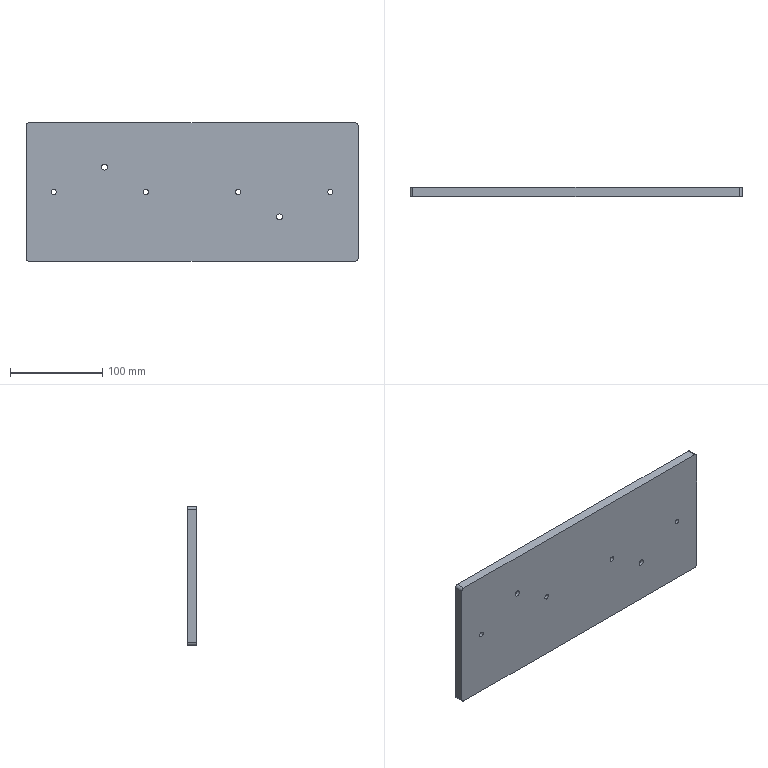Component | SolidWorks | J-006-1 | 1 solid | 40 faces | box 360 x 10 x 150 mm | volume 536326 mm3 | cylinder 28 | plane 12 | commonest cylinder face diameters 10 x8 5.5 x8 11 x4 6.6 x4 6 x4 | material 45
build123d program:
from build123d import *

# Parameters (mm, degrees)
SKETCH1_W                                       = 360
SKETCH1_H                                       = 150
BOSS_EXTRUDE1_DEPTH                             = 10
FILLET1_R                                       = 3
M6_HEX_SOCKET_HEAD_CAP_SCREW_CBORE1_D           = 6.6
M6_HEX_SOCKET_HEAD_CAP_SCREW_CBORE1_CBORE_D     = 11
M6_HEX_SOCKET_HEAD_CAP_SCREW_CBORE1_CBORE_DEPTH = 6.4
M5_HEX_SOCKET_HEAD_CAP_SCREW_CBORE1_D           = 5.5
M5_HEX_SOCKET_HEAD_CAP_SCREW_CBORE1_CBORE_D     = 10
M5_HEX_SOCKET_HEAD_CAP_SCREW_CBORE1_CBORE_DEPTH = 5.4


with BuildPart() as part:
    # Sketch1 → Boss-Extrude1 (new body)
    with BuildSketch(Plane.XY):
        Rectangle(SKETCH1_W, SKETCH1_H)
    extrude(amount=BOSS_EXTRUDE1_DEPTH)

    # Fillet1
    fillet1_edges = [part.edges().sort_by_distance(p)[0] for p in [
        (-180, 75, 5),
        (180, 75, 5),
        (180, -75, 5),
        (-180, -75, 5),
    ]]
    fillet(fillet1_edges, radius=FILLET1_R)

    # M6 Hex Socket Head Cap Screw CBORE1 (through all)
    with Locations(Plane(origin=(0, 0, 0), x_dir=(-1, 0, 0), z_dir=(0, 0, -1))):
        with Locations((-95, -27), (95, 27)):
            CounterBoreHole(M6_HEX_SOCKET_HEAD_CAP_SCREW_CBORE1_D / 2, M6_HEX_SOCKET_HEAD_CAP_SCREW_CBORE1_CBORE_D / 2, M6_HEX_SOCKET_HEAD_CAP_SCREW_CBORE1_CBORE_DEPTH)

    # M5 Hex Socket Head Cap Screw CBORE1 (through all)
    with Locations(Plane(origin=(0, 0, 0), x_dir=(-1, 0, 0), z_dir=(0, 0, -1))):
        with Locations((-150, 0), (-50, 0), (50, 0), (150, 0)):
            CounterBoreHole(M5_HEX_SOCKET_HEAD_CAP_SCREW_CBORE1_D / 2, M5_HEX_SOCKET_HEAD_CAP_SCREW_CBORE1_CBORE_D / 2, M5_HEX_SOCKET_HEAD_CAP_SCREW_CBORE1_CBORE_DEPTH)


solid = part.part

# Placed as in the assembly
solid = solid.moved(Location((220.325, 268.019, 270.731), (90, 0, 0)))